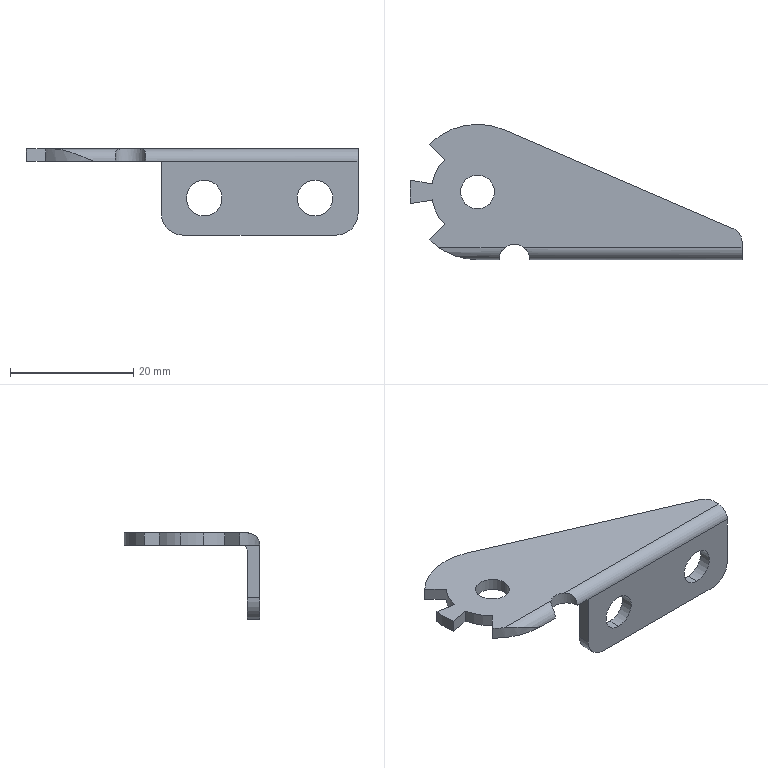Component | SolidWorks | MHPUS204-38-33-A-1_37-1 | 1 solid | 30 faces | box 54 x 22 x 14 mm | volume 2031 mm3 | cylinder 18 | plane 12 | commonest cylinder face diameters 5.8 x4 22 x3 5.5 x2 4 x2 15 x2 7 x2 4.4 x1 5 x1
STEP:
#1=COLOUR_RGB('',0.7922,0.8196,0.9333);
#2=FILL_AREA_STYLE_COLOUR('',#1);
#3=FILL_AREA_STYLE('',(#2));
#4=SURFACE_STYLE_FILL_AREA(#3);
#5=SURFACE_SIDE_STYLE('',(#4));
#6=SURFACE_STYLE_USAGE(.BOTH.,#5);
#7=PRESENTATION_STYLE_ASSIGNMENT((#6));
#8=CARTESIAN_POINT('',(-0.04475,-3.898,3.071));
#9=VERTEX_POINT('',#8);
#10=CARTESIAN_POINT('',(0.1718,-3.898,3.071));
#11=VERTEX_POINT('',#10);
#12=CARTESIAN_POINT('',(0.06352,-3.898,3.071));
#13=DIRECTION('',(0.,0.,1.));
#14=DIRECTION('',(1.,0.,0.));
#15=AXIS2_PLACEMENT_3D('',#12,#13,#14);
#16=CIRCLE('',#15,0.1083);
#17=EDGE_CURVE('',#9,#11,#16,.T.);
#18=ORIENTED_EDGE('',*,*,#17,.F.);
#19=CARTESIAN_POINT('',(-0.04475,-3.898,3.15));
#20=VERTEX_POINT('',#19);
#21=CARTESIAN_POINT('',(-0.04475,-3.898,3.15));
#22=DIRECTION('',(0.,0.,1.));
#23=VECTOR('',#22,39.37);
#24=LINE('',#21,#23);
#25=EDGE_CURVE('',#9,#20,#24,.T.);
#26=ORIENTED_EDGE('',*,*,#25,.T.);
#27=CARTESIAN_POINT('',(0.1718,-3.898,3.15));
#28=VERTEX_POINT('',#27);
#29=CARTESIAN_POINT('',(0.06352,-3.898,3.15));
#30=DIRECTION('',(0.,0.,-1.));
#31=DIRECTION('',(1.,0.,0.));
#32=AXIS2_PLACEMENT_3D('',#29,#30,#31);
#33=CIRCLE('',#32,0.1083);
#34=EDGE_CURVE('',#28,#20,#33,.T.);
#35=ORIENTED_EDGE('',*,*,#34,.F.);
#36=CARTESIAN_POINT('',(0.1718,-3.898,3.15));
#37=DIRECTION('',(0.,0.,1.));
#38=VECTOR('',#37,39.37);
#39=LINE('',#36,#38);
#40=EDGE_CURVE('',#11,#28,#39,.T.);
#41=ORIENTED_EDGE('',*,*,#40,.F.);
#42=EDGE_LOOP('',(#18,#26,#35,#41));
#43=FACE_OUTER_BOUND('',#42,.T.);
#44=CARTESIAN_POINT('',(0.06352,-3.898,3.15));
#45=DIRECTION('',(0.,0.,1.));
#46=DIRECTION('',(1.,0.,0.));
#47=AXIS2_PLACEMENT_3D('',#44,#45,#46);
#48=CYLINDRICAL_SURFACE('',#47,0.1083);
#49=ADVANCED_FACE('',(#43),#48,.F.);
#50=CARTESIAN_POINT('',(0.7722,-4.252,2.72));
#51=VERTEX_POINT('',#50);
#52=CARTESIAN_POINT('',(0.7722,-4.252,2.949));
#53=VERTEX_POINT('',#52);
#54=CARTESIAN_POINT('',(0.7722,-4.252,2.835));
#55=DIRECTION('',(0.,1.,0.));
#56=DIRECTION('',(0.,0.,-1.));
#57=AXIS2_PLACEMENT_3D('',#54,#55,#56);
#58=CIRCLE('',#57,0.1142);
#59=EDGE_CURVE('',#51,#53,#58,.T.);
#60=ORIENTED_EDGE('',*,*,#59,.T.);
#61=CARTESIAN_POINT('',(0.7722,-4.331,2.949));
#62=VERTEX_POINT('',#61);
#63=CARTESIAN_POINT('',(0.7722,-4.331,2.949));
#64=DIRECTION('',(0.,-1.,0.));
#65=VECTOR('',#64,39.37);
#66=LINE('',#63,#65);
#67=EDGE_CURVE('',#53,#62,#66,.T.);
#68=ORIENTED_EDGE('',*,*,#67,.T.);
#69=CARTESIAN_POINT('',(0.7722,-4.331,2.72));
#70=VERTEX_POINT('',#69);
#71=CARTESIAN_POINT('',(0.7722,-4.331,2.835));
#72=DIRECTION('',(0.,1.,0.));
#73=DIRECTION('',(0.,0.,-1.));
#74=AXIS2_PLACEMENT_3D('',#71,#72,#73);
#75=CIRCLE('',#74,0.1142);
#76=EDGE_CURVE('',#70,#62,#75,.T.);
#77=ORIENTED_EDGE('',*,*,#76,.F.);
#78=CARTESIAN_POINT('',(0.7722,-4.331,2.72));
#79=DIRECTION('',(0.,-1.,0.));
#80=VECTOR('',#79,39.37);
#81=LINE('',#78,#80);
#82=EDGE_CURVE('',#51,#70,#81,.T.);
#83=ORIENTED_EDGE('',*,*,#82,.F.);
#84=EDGE_LOOP('',(#60,#68,#77,#83));
#85=FACE_OUTER_BOUND('',#84,.T.);
#86=CARTESIAN_POINT('',(0.7722,-4.331,2.835));
#87=DIRECTION('',(0.,-1.,0.));
#88=DIRECTION('',(0.,0.,-1.));
#89=AXIS2_PLACEMENT_3D('',#86,#87,#88);
#90=CYLINDRICAL_SURFACE('',#89,0.1142);
#91=ADVANCED_FACE('',(#85),#90,.F.);
#92=CARTESIAN_POINT('',(1.481,-4.252,2.72));
#93=VERTEX_POINT('',#92);
#94=CARTESIAN_POINT('',(1.481,-4.252,2.949));
#95=VERTEX_POINT('',#94);
#96=CARTESIAN_POINT('',(1.481,-4.252,2.835));
#97=DIRECTION('',(0.,1.,0.));
#98=DIRECTION('',(0.,0.,-1.));
#99=AXIS2_PLACEMENT_3D('',#96,#97,#98);
#100=CIRCLE('',#99,0.1142);
#101=EDGE_CURVE('',#93,#95,#100,.T.);
#102=ORIENTED_EDGE('',*,*,#101,.T.);
#103=CARTESIAN_POINT('',(1.481,-4.331,2.949));
#104=VERTEX_POINT('',#103);
#105=CARTESIAN_POINT('',(1.481,-4.331,2.949));
#106=DIRECTION('',(0.,-1.,0.));
#107=VECTOR('',#106,39.37);
#108=LINE('',#105,#107);
#109=EDGE_CURVE('',#95,#104,#108,.T.);
#110=ORIENTED_EDGE('',*,*,#109,.T.);
#111=CARTESIAN_POINT('',(1.481,-4.331,2.72));
#112=VERTEX_POINT('',#111);
#113=CARTESIAN_POINT('',(1.481,-4.331,2.835));
#114=DIRECTION('',(0.,1.,0.));
#115=DIRECTION('',(0.,0.,-1.));
#116=AXIS2_PLACEMENT_3D('',#113,#114,#115);
#117=CIRCLE('',#116,0.1142);
#118=EDGE_CURVE('',#112,#104,#117,.T.);
#119=ORIENTED_EDGE('',*,*,#118,.F.);
#120=CARTESIAN_POINT('',(1.481,-4.331,2.72));
#121=DIRECTION('',(0.,-1.,0.));
#122=VECTOR('',#121,39.37);
#123=LINE('',#120,#122);
#124=EDGE_CURVE('',#93,#112,#123,.T.);
#125=ORIENTED_EDGE('',*,*,#124,.F.);
#126=EDGE_LOOP('',(#102,#110,#119,#125));
#127=FACE_OUTER_BOUND('',#126,.T.);
#128=CARTESIAN_POINT('',(1.481,-4.331,2.835));
#129=DIRECTION('',(0.,-1.,0.));
#130=DIRECTION('',(0.,0.,-1.));
#131=AXIS2_PLACEMENT_3D('',#128,#129,#130);
#132=CYLINDRICAL_SURFACE('',#131,0.1142);
#133=ADVANCED_FACE('',(#127),#132,.F.);
#134=ORIENTED_EDGE('',*,*,#34,.T.);
#135=CARTESIAN_POINT('',(0.06352,-3.898,3.15));
#136=DIRECTION('',(0.,0.,-1.));
#137=DIRECTION('',(1.,0.,0.));
#138=AXIS2_PLACEMENT_3D('',#135,#136,#137);
#139=CIRCLE('',#138,0.1083);
#140=EDGE_CURVE('',#20,#28,#139,.T.);
#141=ORIENTED_EDGE('',*,*,#140,.T.);
#142=EDGE_LOOP('',(#134,#141));
#143=FACE_BOUND('',#142,.T.);
#144=CARTESIAN_POINT('',(-0.2427,-4.204,3.15));
#145=VERTEX_POINT('',#144);
#146=CARTESIAN_POINT('',(-0.1855,-4.252,3.15));
#147=VERTEX_POINT('',#146);
#148=CARTESIAN_POINT('',(0.06352,-3.898,3.15));
#149=DIRECTION('',(0.,0.,1.));
#150=DIRECTION('',(1.,0.,0.));
#151=AXIS2_PLACEMENT_3D('',#148,#149,#150);
#152=CIRCLE('',#151,0.4331);
#153=EDGE_CURVE('',#145,#147,#152,.T.);
#154=ORIENTED_EDGE('',*,*,#153,.T.);
#155=CARTESIAN_POINT('',(0.2407,-4.252,3.15));
#156=VERTEX_POINT('',#155);
#157=CARTESIAN_POINT('',(0.06352,-4.252,3.15));
#158=DIRECTION('',(1.,0.,0.));
#159=VECTOR('',#158,39.37);
#160=LINE('',#157,#159);
#161=EDGE_CURVE('',#147,#156,#160,.T.);
#162=ORIENTED_EDGE('',*,*,#161,.T.);
#163=CARTESIAN_POINT('',(0.3588,-4.252,3.15));
#164=VERTEX_POINT('',#163);
#165=CARTESIAN_POINT('',(0.2997,-4.331,3.15));
#166=DIRECTION('',(0.,0.,-1.));
#167=DIRECTION('',(1.,0.,0.));
#168=AXIS2_PLACEMENT_3D('',#165,#166,#167);
#169=CIRCLE('',#168,0.09843);
#170=EDGE_CURVE('',#156,#164,#169,.T.);
#171=ORIENTED_EDGE('',*,*,#170,.T.);
#172=CARTESIAN_POINT('',(1.756,-4.252,3.15));
#173=VERTEX_POINT('',#172);
#174=CARTESIAN_POINT('',(0.06352,-4.252,3.15));
#175=DIRECTION('',(1.,0.,0.));
#176=VECTOR('',#175,39.37);
#177=LINE('',#174,#176);
#178=EDGE_CURVE('',#164,#173,#177,.T.);
#179=ORIENTED_EDGE('',*,*,#178,.T.);
#180=CARTESIAN_POINT('',(1.756,-4.214,3.15));
#181=VERTEX_POINT('',#180);
#182=CARTESIAN_POINT('',(1.756,-4.331,3.15));
#183=DIRECTION('',(0.,-1.,0.));
#184=VECTOR('',#183,39.37);
#185=LINE('',#182,#184);
#186=EDGE_CURVE('',#181,#173,#185,.T.);
#187=ORIENTED_EDGE('',*,*,#186,.F.);
#188=CARTESIAN_POINT('',(1.704,-4.135,3.15));
#189=VERTEX_POINT('',#188);
#190=CARTESIAN_POINT('',(1.67,-4.214,3.15));
#191=DIRECTION('',(0.,0.,1.));
#192=DIRECTION('',(1.,0.,0.));
#193=AXIS2_PLACEMENT_3D('',#190,#191,#192);
#194=CIRCLE('',#193,0.08661);
#195=EDGE_CURVE('',#181,#189,#194,.T.);
#196=ORIENTED_EDGE('',*,*,#195,.T.);
#197=CARTESIAN_POINT('',(0.2353,-3.5,3.15));
#198=VERTEX_POINT('',#197);
#199=CARTESIAN_POINT('',(1.704,-4.135,3.15));
#200=DIRECTION('',(-0.9179,0.3967,0.));
#201=VECTOR('',#200,39.37);
#202=LINE('',#199,#201);
#203=EDGE_CURVE('',#189,#198,#202,.T.);
#204=ORIENTED_EDGE('',*,*,#203,.T.);
#205=CARTESIAN_POINT('',(-0.2427,-3.591,3.15));
#206=VERTEX_POINT('',#205);
#207=CARTESIAN_POINT('',(0.06352,-3.898,3.15));
#208=DIRECTION('',(0.,0.,1.));
#209=DIRECTION('',(1.,0.,0.));
#210=AXIS2_PLACEMENT_3D('',#207,#208,#209);
#211=CIRCLE('',#210,0.4331);
#212=EDGE_CURVE('',#198,#206,#211,.T.);
#213=ORIENTED_EDGE('',*,*,#212,.T.);
#214=CARTESIAN_POINT('',(-0.1453,-3.689,3.15));
#215=VERTEX_POINT('',#214);
#216=CARTESIAN_POINT('',(-0.2427,-3.591,3.15));
#217=DIRECTION('',(0.7071,-0.7071,0.));
#218=VECTOR('',#217,39.37);
#219=LINE('',#216,#218);
#220=EDGE_CURVE('',#206,#215,#219,.T.);
#221=ORIENTED_EDGE('',*,*,#220,.T.);
#222=CARTESIAN_POINT('',(-0.2273,-3.846,3.15));
#223=VERTEX_POINT('',#222);
#224=CARTESIAN_POINT('',(0.06352,-3.898,3.15));
#225=DIRECTION('',(0.,0.,1.));
#226=DIRECTION('',(1.,0.,0.));
#227=AXIS2_PLACEMENT_3D('',#224,#225,#226);
#228=CIRCLE('',#227,0.2953);
#229=EDGE_CURVE('',#215,#223,#228,.T.);
#230=ORIENTED_EDGE('',*,*,#229,.T.);
#231=CARTESIAN_POINT('',(-0.363,-3.822,3.15));
#232=VERTEX_POINT('',#231);
#233=CARTESIAN_POINT('',(-0.2273,-3.846,3.15));
#234=DIRECTION('',(-0.9848,0.1736,0.));
#235=VECTOR('',#234,39.37);
#236=LINE('',#233,#235);
#237=EDGE_CURVE('',#223,#232,#236,.T.);
#238=ORIENTED_EDGE('',*,*,#237,.T.);
#239=CARTESIAN_POINT('',(-0.363,-3.973,3.15));
#240=VERTEX_POINT('',#239);
#241=CARTESIAN_POINT('',(0.06352,-3.898,3.15));
#242=DIRECTION('',(0.,0.,1.));
#243=DIRECTION('',(1.,0.,0.));
#244=AXIS2_PLACEMENT_3D('',#241,#242,#243);
#245=CIRCLE('',#244,0.4331);
#246=EDGE_CURVE('',#232,#240,#245,.T.);
#247=ORIENTED_EDGE('',*,*,#246,.T.);
#248=CARTESIAN_POINT('',(-0.2273,-3.949,3.15));
#249=VERTEX_POINT('',#248);
#250=CARTESIAN_POINT('',(-0.363,-3.973,3.15));
#251=DIRECTION('',(0.9848,0.1736,0.));
#252=VECTOR('',#251,39.37);
#253=LINE('',#250,#252);
#254=EDGE_CURVE('',#240,#249,#253,.T.);
#255=ORIENTED_EDGE('',*,*,#254,.T.);
#256=CARTESIAN_POINT('',(-0.1453,-4.106,3.15));
#257=VERTEX_POINT('',#256);
#258=CARTESIAN_POINT('',(0.06352,-3.898,3.15));
#259=DIRECTION('',(0.,0.,1.));
#260=DIRECTION('',(1.,0.,0.));
#261=AXIS2_PLACEMENT_3D('',#258,#259,#260);
#262=CIRCLE('',#261,0.2953);
#263=EDGE_CURVE('',#249,#257,#262,.T.);
#264=ORIENTED_EDGE('',*,*,#263,.T.);
#265=CARTESIAN_POINT('',(-0.1453,-4.106,3.15));
#266=DIRECTION('',(-0.7071,-0.7071,0.));
#267=VECTOR('',#266,39.37);
#268=LINE('',#265,#267);
#269=EDGE_CURVE('',#257,#145,#268,.T.);
#270=ORIENTED_EDGE('',*,*,#269,.T.);
#271=EDGE_LOOP('',(#154,#162,#171,#179,#187,#196,#204,#213,#221,#230,#238,#247,#255,#264,#270));
#272=FACE_OUTER_BOUND('',#271,.T.);
#273=CARTESIAN_POINT('',(0.06352,-4.331,3.15));
#274=DIRECTION('',(0.,0.,1.));
#275=DIRECTION('',(1.,0.,0.));
#276=AXIS2_PLACEMENT_3D('',#273,#274,#275);
#277=PLANE('',#276);
#278=ADVANCED_FACE('',(#143,#272),#277,.T.);
#279=ORIENTED_EDGE('',*,*,#25,.F.);
#280=CARTESIAN_POINT('',(0.06352,-3.898,3.071));
#281=DIRECTION('',(0.,0.,1.));
#282=DIRECTION('',(1.,0.,0.));
#283=AXIS2_PLACEMENT_3D('',#280,#281,#282);
#284=CIRCLE('',#283,0.1083);
#285=EDGE_CURVE('',#11,#9,#284,.T.);
#286=ORIENTED_EDGE('',*,*,#285,.F.);
#287=ORIENTED_EDGE('',*,*,#40,.T.);
#288=ORIENTED_EDGE('',*,*,#140,.F.);
#289=EDGE_LOOP('',(#279,#286,#287,#288));
#290=FACE_OUTER_BOUND('',#289,.T.);
#291=CARTESIAN_POINT('',(0.06352,-3.898,3.15));
#292=DIRECTION('',(0.,0.,1.));
#293=DIRECTION('',(1.,0.,0.));
#294=AXIS2_PLACEMENT_3D('',#291,#292,#293);
#295=CYLINDRICAL_SURFACE('',#294,0.1083);
#296=ADVANCED_FACE('',(#290),#295,.F.);
#297=CARTESIAN_POINT('',(0.06352,-4.331,3.071));
#298=VERTEX_POINT('',#297);
#299=CARTESIAN_POINT('',(-0.1855,-4.252,3.15));
#300=CARTESIAN_POINT('',(-0.1663,-4.265,3.15));
#301=CARTESIAN_POINT('',(-0.1465,-4.277,3.146));
#302=CARTESIAN_POINT('',(-0.1158,-4.292,3.139));
#303=CARTESIAN_POINT('',(-0.1054,-4.297,3.136));
#304=CARTESIAN_POINT('',(-0.08469,-4.305,3.13));
#305=CARTESIAN_POINT('',(-0.0743,-4.308,3.126));
#306=CARTESIAN_POINT('',(-0.04301,-4.318,3.115));
#307=CARTESIAN_POINT('',(-0.02197,-4.323,3.107));
#308=CARTESIAN_POINT('',(0.01002,-4.328,3.094));
#309=CARTESIAN_POINT('',(0.02072,-4.329,3.089));
#310=CARTESIAN_POINT('',(0.0421,-4.33,3.08));
#311=CARTESIAN_POINT('',(0.05286,-4.331,3.075));
#312=CARTESIAN_POINT('',(0.06352,-4.331,3.071));
#313=B_SPLINE_CURVE_WITH_KNOTS('',3,(#299,#300,#301,#302,#303,#304,#305,#306,#307,#308,#309,#310,#311,#312),.UNSPECIFIED.,.F.,.F.,(4,2,2,2,2,2,4),(0.,0.001765,0.002648,0.003531,0.005296,0.006179,0.007061),.UNSPECIFIED.);
#314=EDGE_CURVE('',#147,#298,#313,.T.);
#315=ORIENTED_EDGE('',*,*,#314,.T.);
#316=CARTESIAN_POINT('',(0.2013,-4.331,3.071));
#317=VERTEX_POINT('',#316);
#318=CARTESIAN_POINT('',(1.756,-4.331,3.071));
#319=DIRECTION('',(1.,0.,0.));
#320=VECTOR('',#319,39.37);
#321=LINE('',#318,#320);
#322=EDGE_CURVE('',#298,#317,#321,.T.);
#323=ORIENTED_EDGE('',*,*,#322,.T.);
#324=CARTESIAN_POINT('',(0.2013,-4.331,3.071));
#325=CARTESIAN_POINT('',(0.2013,-4.331,3.077));
#326=CARTESIAN_POINT('',(0.2013,-4.33,3.082));
#327=CARTESIAN_POINT('',(0.2013,-4.328,3.093));
#328=CARTESIAN_POINT('',(0.2014,-4.326,3.099));
#329=CARTESIAN_POINT('',(0.2017,-4.321,3.109));
#330=CARTESIAN_POINT('',(0.202,-4.318,3.114));
#331=CARTESIAN_POINT('',(0.2031,-4.311,3.123));
#332=CARTESIAN_POINT('',(0.204,-4.308,3.127));
#333=CARTESIAN_POINT('',(0.2063,-4.299,3.134));
#334=CARTESIAN_POINT('',(0.208,-4.295,3.137));
#335=CARTESIAN_POINT('',(0.2121,-4.286,3.142));
#336=CARTESIAN_POINT('',(0.2146,-4.281,3.144));
#337=CARTESIAN_POINT('',(0.2237,-4.267,3.149));
#338=CARTESIAN_POINT('',(0.2316,-4.259,3.15));
#339=CARTESIAN_POINT('',(0.2407,-4.252,3.15));
#340=B_SPLINE_CURVE_WITH_KNOTS('',3,(#324,#325,#326,#327,#328,#329,#330,#331,#332,#333,#334,#335,#336,#337,#338,#339),.UNSPECIFIED.,.F.,.F.,(4,2,2,2,2,2,2,4),(0.,0.0004284,0.0008569,0.001285,0.001714,0.002142,0.002571,0.003428),.UNSPECIFIED.);
#341=EDGE_CURVE('',#317,#156,#340,.T.);
#342=ORIENTED_EDGE('',*,*,#341,.T.);
#343=ORIENTED_EDGE('',*,*,#161,.F.);
#344=EDGE_LOOP('',(#315,#323,#342,#343));
#345=FACE_OUTER_BOUND('',#344,.T.);
#346=CARTESIAN_POINT('',(1.756,-4.252,3.071));
#347=DIRECTION('',(1.,0.,0.));
#348=DIRECTION('',(0.,0.,-1.));
#349=AXIS2_PLACEMENT_3D('',#346,#347,#348);
#350=CYLINDRICAL_SURFACE('',#349,0.07874);
#351=ADVANCED_FACE('',(#345),#350,.T.);
#352=ORIENTED_EDGE('',*,*,#153,.F.);
#353=CARTESIAN_POINT('',(-0.2427,-4.204,3.071));
#354=VERTEX_POINT('',#353);
#355=CARTESIAN_POINT('',(-0.2427,-4.204,3.15));
#356=DIRECTION('',(0.,0.,-1.));
#357=VECTOR('',#356,39.37);
#358=LINE('',#355,#357);
#359=EDGE_CURVE('',#145,#354,#358,.T.);
#360=ORIENTED_EDGE('',*,*,#359,.T.);
#361=CARTESIAN_POINT('',(0.06352,-3.898,3.071));
#362=DIRECTION('',(0.,0.,1.));
#363=DIRECTION('',(1.,0.,0.));
#364=AXIS2_PLACEMENT_3D('',#361,#362,#363);
#365=CIRCLE('',#364,0.4331);
#366=EDGE_CURVE('',#354,#298,#365,.T.);
#367=ORIENTED_EDGE('',*,*,#366,.T.);
#368=ORIENTED_EDGE('',*,*,#314,.F.);
#369=EDGE_LOOP('',(#352,#360,#367,#368));
#370=FACE_OUTER_BOUND('',#369,.T.);
#371=CARTESIAN_POINT('',(0.06352,-3.898,3.15));
#372=DIRECTION('',(0.,0.,1.));
#373=DIRECTION('',(1.,0.,0.));
#374=AXIS2_PLACEMENT_3D('',#371,#372,#373);
#375=CYLINDRICAL_SURFACE('',#374,0.4331);
#376=ADVANCED_FACE('',(#370),#375,.T.);
#377=ORIENTED_EDGE('',*,*,#269,.F.);
#378=CARTESIAN_POINT('',(-0.1453,-4.106,3.071));
#379=VERTEX_POINT('',#378);
#380=CARTESIAN_POINT('',(-0.1453,-4.106,3.15));
#381=DIRECTION('',(0.,0.,-1.));
#382=VECTOR('',#381,39.37);
#383=LINE('',#380,#382);
#384=EDGE_CURVE('',#257,#379,#383,.T.);
#385=ORIENTED_EDGE('',*,*,#384,.T.);
#386=CARTESIAN_POINT('',(-0.1453,-4.106,3.071));
#387=DIRECTION('',(-0.7071,-0.7071,0.));
#388=VECTOR('',#387,39.37);
#389=LINE('',#386,#388);
#390=EDGE_CURVE('',#379,#354,#389,.T.);
#391=ORIENTED_EDGE('',*,*,#390,.T.);
#392=ORIENTED_EDGE('',*,*,#359,.F.);
#393=EDGE_LOOP('',(#377,#385,#391,#392));
#394=FACE_OUTER_BOUND('',#393,.T.);
#395=CARTESIAN_POINT('',(-0.1453,-4.106,3.15));
#396=DIRECTION('',(-0.7071,0.7071,0.));
#397=DIRECTION('',(-0.7071,-0.7071,0.));
#398=AXIS2_PLACEMENT_3D('',#395,#396,#397);
#399=PLANE('',#398);
#400=ADVANCED_FACE('',(#394),#399,.T.);
#401=ORIENTED_EDGE('',*,*,#263,.F.);
#402=CARTESIAN_POINT('',(-0.2273,-3.949,3.071));
#403=VERTEX_POINT('',#402);
#404=CARTESIAN_POINT('',(-0.2273,-3.949,3.15));
#405=DIRECTION('',(0.,0.,-1.));
#406=VECTOR('',#405,39.37);
#407=LINE('',#404,#406);
#408=EDGE_CURVE('',#249,#403,#407,.T.);
#409=ORIENTED_EDGE('',*,*,#408,.T.);
#410=CARTESIAN_POINT('',(0.06352,-3.898,3.071));
#411=DIRECTION('',(0.,0.,1.));
#412=DIRECTION('',(1.,0.,0.));
#413=AXIS2_PLACEMENT_3D('',#410,#411,#412);
#414=CIRCLE('',#413,0.2953);
#415=EDGE_CURVE('',#403,#379,#414,.T.);
#416=ORIENTED_EDGE('',*,*,#415,.T.);
#417=ORIENTED_EDGE('',*,*,#384,.F.);
#418=EDGE_LOOP('',(#401,#409,#416,#417));
#419=FACE_OUTER_BOUND('',#418,.T.);
#420=CARTESIAN_POINT('',(0.06352,-3.898,3.15));
#421=DIRECTION('',(0.,0.,1.));
#422=DIRECTION('',(1.,0.,0.));
#423=AXIS2_PLACEMENT_3D('',#420,#421,#422);
#424=CYLINDRICAL_SURFACE('',#423,0.2953);
#425=ADVANCED_FACE('',(#419),#424,.T.);
#426=ORIENTED_EDGE('',*,*,#254,.F.);
#427=CARTESIAN_POINT('',(-0.363,-3.973,3.071));
#428=VERTEX_POINT('',#427);
#429=CARTESIAN_POINT('',(-0.363,-3.973,3.15));
#430=DIRECTION('',(0.,0.,-1.));
#431=VECTOR('',#430,39.37);
#432=LINE('',#429,#431);
#433=EDGE_CURVE('',#240,#428,#432,.T.);
#434=ORIENTED_EDGE('',*,*,#433,.T.);
#435=CARTESIAN_POINT('',(-0.363,-3.973,3.071));
#436=DIRECTION('',(0.9848,0.1736,0.));
#437=VECTOR('',#436,39.37);
#438=LINE('',#435,#437);
#439=EDGE_CURVE('',#428,#403,#438,.T.);
#440=ORIENTED_EDGE('',*,*,#439,.T.);
#441=ORIENTED_EDGE('',*,*,#408,.F.);
#442=EDGE_LOOP('',(#426,#434,#440,#441));
#443=FACE_OUTER_BOUND('',#442,.T.);
#444=CARTESIAN_POINT('',(-0.363,-3.973,3.15));
#445=DIRECTION('',(0.1736,-0.9848,0.));
#446=DIRECTION('',(0.9848,0.1736,0.));
#447=AXIS2_PLACEMENT_3D('',#444,#445,#446);
#448=PLANE('',#447);
#449=ADVANCED_FACE('',(#443),#448,.T.);
#450=ORIENTED_EDGE('',*,*,#246,.F.);
#451=CARTESIAN_POINT('',(-0.363,-3.822,3.071));
#452=VERTEX_POINT('',#451);
#453=CARTESIAN_POINT('',(-0.363,-3.822,3.15));
#454=DIRECTION('',(0.,0.,-1.));
#455=VECTOR('',#454,39.37);
#456=LINE('',#453,#455);
#457=EDGE_CURVE('',#232,#452,#456,.T.);
#458=ORIENTED_EDGE('',*,*,#457,.T.);
#459=CARTESIAN_POINT('',(0.06352,-3.898,3.071));
#460=DIRECTION('',(0.,0.,1.));
#461=DIRECTION('',(1.,0.,0.));
#462=AXIS2_PLACEMENT_3D('',#459,#460,#461);
#463=CIRCLE('',#462,0.4331);
#464=EDGE_CURVE('',#452,#428,#463,.T.);
#465=ORIENTED_EDGE('',*,*,#464,.T.);
#466=ORIENTED_EDGE('',*,*,#433,.F.);
#467=EDGE_LOOP('',(#450,#458,#465,#466));
#468=FACE_OUTER_BOUND('',#467,.T.);
#469=CARTESIAN_POINT('',(0.06352,-3.898,3.15));
#470=DIRECTION('',(0.,0.,1.));
#471=DIRECTION('',(1.,0.,0.));
#472=AXIS2_PLACEMENT_3D('',#469,#470,#471);
#473=CYLINDRICAL_SURFACE('',#472,0.4331);
#474=ADVANCED_FACE('',(#468),#473,.T.);
#475=ORIENTED_EDGE('',*,*,#237,.F.);
#476=CARTESIAN_POINT('',(-0.2273,-3.846,3.071));
#477=VERTEX_POINT('',#476);
#478=CARTESIAN_POINT('',(-0.2273,-3.846,3.15));
#479=DIRECTION('',(0.,0.,-1.));
#480=VECTOR('',#479,39.37);
#481=LINE('',#478,#480);
#482=EDGE_CURVE('',#223,#477,#481,.T.);
#483=ORIENTED_EDGE('',*,*,#482,.T.);
#484=CARTESIAN_POINT('',(-0.2273,-3.846,3.071));
#485=DIRECTION('',(-0.9848,0.1736,0.));
#486=VECTOR('',#485,39.37);
#487=LINE('',#484,#486);
#488=EDGE_CURVE('',#477,#452,#487,.T.);
#489=ORIENTED_EDGE('',*,*,#488,.T.);
#490=ORIENTED_EDGE('',*,*,#457,.F.);
#491=EDGE_LOOP('',(#475,#483,#489,#490));
#492=FACE_OUTER_BOUND('',#491,.T.);
#493=CARTESIAN_POINT('',(-0.2273,-3.846,3.15));
#494=DIRECTION('',(0.1736,0.9848,0.));
#495=DIRECTION('',(-0.9848,0.1736,0.));
#496=AXIS2_PLACEMENT_3D('',#493,#494,#495);
#497=PLANE('',#496);
#498=ADVANCED_FACE('',(#492),#497,.T.);
#499=ORIENTED_EDGE('',*,*,#229,.F.);
#500=CARTESIAN_POINT('',(-0.1453,-3.689,3.071));
#501=VERTEX_POINT('',#500);
#502=CARTESIAN_POINT('',(-0.1453,-3.689,3.15));
#503=DIRECTION('',(0.,0.,-1.));
#504=VECTOR('',#503,39.37);
#505=LINE('',#502,#504);
#506=EDGE_CURVE('',#215,#501,#505,.T.);
#507=ORIENTED_EDGE('',*,*,#506,.T.);
#508=CARTESIAN_POINT('',(0.06352,-3.898,3.071));
#509=DIRECTION('',(0.,0.,1.));
#510=DIRECTION('',(1.,0.,0.));
#511=AXIS2_PLACEMENT_3D('',#508,#509,#510);
#512=CIRCLE('',#511,0.2953);
#513=EDGE_CURVE('',#501,#477,#512,.T.);
#514=ORIENTED_EDGE('',*,*,#513,.T.);
#515=ORIENTED_EDGE('',*,*,#482,.F.);
#516=EDGE_LOOP('',(#499,#507,#514,#515));
#517=FACE_OUTER_BOUND('',#516,.T.);
#518=CARTESIAN_POINT('',(0.06352,-3.898,3.15));
#519=DIRECTION('',(0.,0.,1.));
#520=DIRECTION('',(1.,0.,0.));
#521=AXIS2_PLACEMENT_3D('',#518,#519,#520);
#522=CYLINDRICAL_SURFACE('',#521,0.2953);
#523=ADVANCED_FACE('',(#517),#522,.T.);
#524=ORIENTED_EDGE('',*,*,#220,.F.);
#525=CARTESIAN_POINT('',(-0.2427,-3.591,3.071));
#526=VERTEX_POINT('',#525);
#527=CARTESIAN_POINT('',(-0.2427,-3.591,3.15));
#528=DIRECTION('',(0.,0.,-1.));
#529=VECTOR('',#528,39.37);
#530=LINE('',#527,#529);
#531=EDGE_CURVE('',#206,#526,#530,.T.);
#532=ORIENTED_EDGE('',*,*,#531,.T.);
#533=CARTESIAN_POINT('',(-0.2427,-3.591,3.071));
#534=DIRECTION('',(0.7071,-0.7071,0.));
#535=VECTOR('',#534,39.37);
#536=LINE('',#533,#535);
#537=EDGE_CURVE('',#526,#501,#536,.T.);
#538=ORIENTED_EDGE('',*,*,#537,.T.);
#539=ORIENTED_EDGE('',*,*,#506,.F.);
#540=EDGE_LOOP('',(#524,#532,#538,#539));
#541=FACE_OUTER_BOUND('',#540,.T.);
#542=CARTESIAN_POINT('',(-0.2427,-3.591,3.15));
#543=DIRECTION('',(-0.7071,-0.7071,0.));
#544=DIRECTION('',(0.7071,-0.7071,0.));
#545=AXIS2_PLACEMENT_3D('',#542,#543,#544);
#546=PLANE('',#545);
#547=ADVANCED_FACE('',(#541),#546,.T.);
#548=ORIENTED_EDGE('',*,*,#212,.F.);
#549=CARTESIAN_POINT('',(0.2353,-3.5,3.071));
#550=VERTEX_POINT('',#549);
#551=CARTESIAN_POINT('',(0.2353,-3.5,3.15));
#552=DIRECTION('',(0.,0.,-1.));
#553=VECTOR('',#552,39.37);
#554=LINE('',#551,#553);
#555=EDGE_CURVE('',#198,#550,#554,.T.);
#556=ORIENTED_EDGE('',*,*,#555,.T.);
#557=CARTESIAN_POINT('',(0.06352,-3.898,3.071));
#558=DIRECTION('',(0.,0.,1.));
#559=DIRECTION('',(1.,0.,0.));
#560=AXIS2_PLACEMENT_3D('',#557,#558,#559);
#561=CIRCLE('',#560,0.4331);
#562=EDGE_CURVE('',#550,#526,#561,.T.);
#563=ORIENTED_EDGE('',*,*,#562,.T.);
#564=ORIENTED_EDGE('',*,*,#531,.F.);
#565=EDGE_LOOP('',(#548,#556,#563,#564));
#566=FACE_OUTER_BOUND('',#565,.T.);
#567=CARTESIAN_POINT('',(0.06352,-3.898,3.15));
#568=DIRECTION('',(0.,0.,1.));
#569=DIRECTION('',(1.,0.,0.));
#570=AXIS2_PLACEMENT_3D('',#567,#568,#569);
#571=CYLINDRICAL_SURFACE('',#570,0.4331);
#572=ADVANCED_FACE('',(#566),#571,.T.);
#573=ORIENTED_EDGE('',*,*,#203,.F.);
#574=CARTESIAN_POINT('',(1.704,-4.135,3.071));
#575=VERTEX_POINT('',#574);
#576=CARTESIAN_POINT('',(1.704,-4.135,3.15));
#577=DIRECTION('',(0.,0.,-1.));
#578=VECTOR('',#577,39.37);
#579=LINE('',#576,#578);
#580=EDGE_CURVE('',#189,#575,#579,.T.);
#581=ORIENTED_EDGE('',*,*,#580,.T.);
#582=CARTESIAN_POINT('',(1.704,-4.135,3.071));
#583=DIRECTION('',(-0.9179,0.3967,0.));
#584=VECTOR('',#583,39.37);
#585=LINE('',#582,#584);
#586=EDGE_CURVE('',#575,#550,#585,.T.);
#587=ORIENTED_EDGE('',*,*,#586,.T.);
#588=ORIENTED_EDGE('',*,*,#555,.F.);
#589=EDGE_LOOP('',(#573,#581,#587,#588));
#590=FACE_OUTER_BOUND('',#589,.T.);
#591=CARTESIAN_POINT('',(1.704,-4.135,3.15));
#592=DIRECTION('',(0.3967,0.9179,0.));
#593=DIRECTION('',(-0.9179,0.3967,0.));
#594=AXIS2_PLACEMENT_3D('',#591,#592,#593);
#595=PLANE('',#594);
#596=ADVANCED_FACE('',(#590),#595,.T.);
#597=ORIENTED_EDGE('',*,*,#195,.F.);
#598=CARTESIAN_POINT('',(1.756,-4.214,3.071));
#599=VERTEX_POINT('',#598);
#600=CARTESIAN_POINT('',(1.756,-4.214,3.15));
#601=DIRECTION('',(0.,0.,-1.));
#602=VECTOR('',#601,39.37);
#603=LINE('',#600,#602);
#604=EDGE_CURVE('',#181,#599,#603,.T.);
#605=ORIENTED_EDGE('',*,*,#604,.T.);
#606=CARTESIAN_POINT('',(1.756,-4.213,3.071));
#607=VERTEX_POINT('',#606);
#608=CARTESIAN_POINT('',(1.756,-4.214,3.071));
#609=CARTESIAN_POINT('',(1.756,-4.214,3.071));
#610=CARTESIAN_POINT('',(1.756,-4.213,3.071));
#611=CARTESIAN_POINT('',(1.756,-4.213,3.071));
#612=B_SPLINE_CURVE_WITH_KNOTS('',3,(#608,#609,#610,#611),.UNSPECIFIED.,.F.,.F.,(4,4),(0.,0.0000459),.UNSPECIFIED.);
#613=EDGE_CURVE('',#599,#607,#612,.T.);
#614=ORIENTED_EDGE('',*,*,#613,.T.);
#615=CARTESIAN_POINT('',(1.67,-4.214,3.071));
#616=DIRECTION('',(0.,0.,1.));
#617=DIRECTION('',(1.,0.,0.));
#618=AXIS2_PLACEMENT_3D('',#615,#616,#617);
#619=CIRCLE('',#618,0.08661);
#620=EDGE_CURVE('',#607,#575,#619,.T.);
#621=ORIENTED_EDGE('',*,*,#620,.T.);
#622=ORIENTED_EDGE('',*,*,#580,.F.);
#623=EDGE_LOOP('',(#597,#605,#614,#621,#622));
#624=FACE_OUTER_BOUND('',#623,.T.);
#625=CARTESIAN_POINT('',(1.67,-4.214,3.15));
#626=DIRECTION('',(0.,0.,1.));
#627=DIRECTION('',(1.,0.,0.));
#628=AXIS2_PLACEMENT_3D('',#625,#626,#627);
#629=CYLINDRICAL_SURFACE('',#628,0.08661);
#630=ADVANCED_FACE('',(#624),#629,.T.);
#631=CARTESIAN_POINT('',(1.756,-4.331,3.071));
#632=VERTEX_POINT('',#631);
#633=CARTESIAN_POINT('',(1.756,-4.252,3.071));
#634=DIRECTION('',(-1.,0.,0.));
#635=DIRECTION('',(0.,0.,-1.));
#636=AXIS2_PLACEMENT_3D('',#633,#634,#635);
#637=CIRCLE('',#636,0.07874);
#638=EDGE_CURVE('',#632,#173,#637,.T.);
#639=ORIENTED_EDGE('',*,*,#638,.T.);
#640=ORIENTED_EDGE('',*,*,#178,.F.);
#641=CARTESIAN_POINT('',(0.3982,-4.331,3.071));
#642=VERTEX_POINT('',#641);
#643=CARTESIAN_POINT('',(0.3588,-4.252,3.15));
#644=CARTESIAN_POINT('',(0.3633,-4.255,3.15));
#645=CARTESIAN_POINT('',(0.3675,-4.259,3.149));
#646=CARTESIAN_POINT('',(0.3752,-4.267,3.148));
#647=CARTESIAN_POINT('',(0.3787,-4.272,3.147));
#648=CARTESIAN_POINT('',(0.3847,-4.281,3.144));
#649=CARTESIAN_POINT('',(0.3873,-4.285,3.142));
#650=CARTESIAN_POINT('',(0.3915,-4.295,3.137));
#651=CARTESIAN_POINT('',(0.3931,-4.299,3.134));
#652=CARTESIAN_POINT('',(0.3955,-4.307,3.127));
#653=CARTESIAN_POINT('',(0.3963,-4.311,3.123));
#654=CARTESIAN_POINT('',(0.3974,-4.318,3.114));
#655=CARTESIAN_POINT('',(0.3977,-4.321,3.109));
#656=CARTESIAN_POINT('',(0.3981,-4.326,3.099));
#657=CARTESIAN_POINT('',(0.3981,-4.328,3.093));
#658=CARTESIAN_POINT('',(0.3982,-4.33,3.082));
#659=CARTESIAN_POINT('',(0.3982,-4.331,3.077));
#660=CARTESIAN_POINT('',(0.3982,-4.331,3.071));
#661=B_SPLINE_CURVE_WITH_KNOTS('',3,(#643,#644,#645,#646,#647,#648,#649,#650,#651,#652,#653,#654,#655,#656,#657,#658,#659,#660),.UNSPECIFIED.,.F.,.F.,(4,2,2,2,2,2,2,2,4),(0.,0.0004287,0.0008574,0.001286,0.001715,0.002144,0.002572,0.003001,0.00343),.UNSPECIFIED.);
#662=EDGE_CURVE('',#164,#642,#661,.T.);
#663=ORIENTED_EDGE('',*,*,#662,.T.);
#664=CARTESIAN_POINT('',(0.4966,-4.331,3.071));
#665=VERTEX_POINT('',#664);
#666=CARTESIAN_POINT('',(1.756,-4.331,3.071));
#667=DIRECTION('',(1.,0.,0.));
#668=VECTOR('',#667,39.37);
#669=LINE('',#666,#668);
#670=EDGE_CURVE('',#642,#665,#669,.T.);
#671=ORIENTED_EDGE('',*,*,#670,.T.);
#672=CARTESIAN_POINT('',(1.756,-4.331,3.071));
#673=DIRECTION('',(1.,0.,0.));
#674=VECTOR('',#673,39.37);
#675=LINE('',#672,#674);
#676=EDGE_CURVE('',#665,#632,#675,.T.);
#677=ORIENTED_EDGE('',*,*,#676,.T.);
#678=EDGE_LOOP('',(#639,#640,#663,#671,#677));
#679=FACE_OUTER_BOUND('',#678,.T.);
#680=CARTESIAN_POINT('',(1.756,-4.252,3.071));
#681=DIRECTION('',(1.,0.,0.));
#682=DIRECTION('',(0.,0.,-1.));
#683=AXIS2_PLACEMENT_3D('',#680,#681,#682);
#684=CYLINDRICAL_SURFACE('',#683,0.07874);
#685=ADVANCED_FACE('',(#679),#684,.T.);
#686=ORIENTED_EDGE('',*,*,#170,.F.);
#687=ORIENTED_EDGE('',*,*,#341,.F.);
#688=CARTESIAN_POINT('',(0.2997,-4.331,3.071));
#689=DIRECTION('',(0.,0.,1.));
#690=DIRECTION('',(1.,0.,0.));
#691=AXIS2_PLACEMENT_3D('',#688,#689,#690);
#692=CIRCLE('',#691,0.09843);
#693=EDGE_CURVE('',#642,#317,#692,.T.);
#694=ORIENTED_EDGE('',*,*,#693,.F.);
#695=ORIENTED_EDGE('',*,*,#662,.F.);
#696=EDGE_LOOP('',(#686,#687,#694,#695));
#697=FACE_OUTER_BOUND('',#696,.T.);
#698=CARTESIAN_POINT('',(0.2997,-4.331,3.15));
#699=DIRECTION('',(0.,0.,1.));
#700=DIRECTION('',(1.,0.,0.));
#701=AXIS2_PLACEMENT_3D('',#698,#699,#700);
#702=CYLINDRICAL_SURFACE('',#701,0.09843);
#703=ADVANCED_FACE('',(#697),#702,.F.);
#704=ORIENTED_EDGE('',*,*,#285,.T.);
#705=ORIENTED_EDGE('',*,*,#17,.T.);
#706=EDGE_LOOP('',(#704,#705));
#707=FACE_BOUND('',#706,.T.);
#708=ORIENTED_EDGE('',*,*,#322,.F.);
#709=ORIENTED_EDGE('',*,*,#366,.F.);
#710=ORIENTED_EDGE('',*,*,#390,.F.);
#711=ORIENTED_EDGE('',*,*,#415,.F.);
#712=ORIENTED_EDGE('',*,*,#439,.F.);
#713=ORIENTED_EDGE('',*,*,#464,.F.);
#714=ORIENTED_EDGE('',*,*,#488,.F.);
#715=ORIENTED_EDGE('',*,*,#513,.F.);
#716=ORIENTED_EDGE('',*,*,#537,.F.);
#717=ORIENTED_EDGE('',*,*,#562,.F.);
#718=ORIENTED_EDGE('',*,*,#586,.F.);
#719=ORIENTED_EDGE('',*,*,#620,.F.);
#720=CARTESIAN_POINT('',(0.4966,-4.213,3.071));
#721=VERTEX_POINT('',#720);
#722=CARTESIAN_POINT('',(1.756,-4.213,3.071));
#723=DIRECTION('',(1.,0.,0.));
#724=VECTOR('',#723,39.37);
#725=LINE('',#722,#724);
#726=EDGE_CURVE('',#721,#607,#725,.T.);
#727=ORIENTED_EDGE('',*,*,#726,.F.);
#728=CARTESIAN_POINT('',(0.4966,-3.465,3.071));
#729=DIRECTION('',(0.,1.,0.));
#730=VECTOR('',#729,39.37);
#731=LINE('',#728,#730);
#732=EDGE_CURVE('',#665,#721,#731,.T.);
#733=ORIENTED_EDGE('',*,*,#732,.F.);
#734=ORIENTED_EDGE('',*,*,#670,.F.);
#735=ORIENTED_EDGE('',*,*,#693,.T.);
#736=EDGE_LOOP('',(#708,#709,#710,#711,#712,#713,#714,#715,#716,#717,#718,#719,#727,#733,#734,#735));
#737=FACE_OUTER_BOUND('',#736,.T.);
#738=CARTESIAN_POINT('',(1.756,-3.465,3.071));
#739=DIRECTION('',(0.,0.,1.));
#740=DIRECTION('',(1.,0.,0.));
#741=AXIS2_PLACEMENT_3D('',#738,#739,#740);
#742=PLANE('',#741);
#743=ADVANCED_FACE('',(#707,#737),#742,.F.);
#744=ORIENTED_EDGE('',*,*,#638,.F.);
#745=CARTESIAN_POINT('',(1.756,-4.331,2.736));
#746=VERTEX_POINT('',#745);
#747=CARTESIAN_POINT('',(1.756,-4.331,3.15));
#748=DIRECTION('',(0.,0.,-1.));
#749=VECTOR('',#748,39.37);
#750=LINE('',#747,#749);
#751=EDGE_CURVE('',#632,#746,#750,.T.);
#752=ORIENTED_EDGE('',*,*,#751,.T.);
#753=CARTESIAN_POINT('',(1.756,-4.252,2.736));
#754=VERTEX_POINT('',#753);
#755=CARTESIAN_POINT('',(1.756,-4.331,2.736));
#756=DIRECTION('',(0.,1.,0.));
#757=VECTOR('',#756,39.37);
#758=LINE('',#755,#757);
#759=EDGE_CURVE('',#746,#754,#758,.T.);
#760=ORIENTED_EDGE('',*,*,#759,.T.);
#761=CARTESIAN_POINT('',(1.756,-4.252,3.031));
#762=VERTEX_POINT('',#761);
#763=CARTESIAN_POINT('',(1.756,-4.252,3.15));
#764=DIRECTION('',(0.,0.,1.));
#765=VECTOR('',#764,39.37);
#766=LINE('',#763,#765);
#767=EDGE_CURVE('',#754,#762,#766,.T.);
#768=ORIENTED_EDGE('',*,*,#767,.T.);
#769=CARTESIAN_POINT('',(1.756,-4.213,3.031));
#770=DIRECTION('',(-1.,0.,0.));
#771=DIRECTION('',(0.,0.,-1.));
#772=AXIS2_PLACEMENT_3D('',#769,#770,#771);
#773=CIRCLE('',#772,0.03937);
#774=EDGE_CURVE('',#762,#599,#773,.T.);
#775=ORIENTED_EDGE('',*,*,#774,.T.);
#776=ORIENTED_EDGE('',*,*,#604,.F.);
#777=ORIENTED_EDGE('',*,*,#186,.T.);
#778=EDGE_LOOP('',(#744,#752,#760,#768,#775,#776,#777));
#779=FACE_OUTER_BOUND('',#778,.T.);
#780=CARTESIAN_POINT('',(1.756,-4.331,3.15));
#781=DIRECTION('',(1.,0.,0.));
#782=DIRECTION('',(0.,0.,-1.));
#783=AXIS2_PLACEMENT_3D('',#780,#781,#782);
#784=PLANE('',#783);
#785=ADVANCED_FACE('',(#779),#784,.T.);
#786=CARTESIAN_POINT('',(0.4966,-4.331,2.736));
#787=VERTEX_POINT('',#786);
#788=CARTESIAN_POINT('',(0.6344,-4.331,2.598));
#789=VERTEX_POINT('',#788);
#790=CARTESIAN_POINT('',(0.6344,-4.331,2.736));
#791=DIRECTION('',(0.,-1.,0.));
#792=DIRECTION('',(0.,0.,-1.));
#793=AXIS2_PLACEMENT_3D('',#790,#791,#792);
#794=CIRCLE('',#793,0.1378);
#795=EDGE_CURVE('',#787,#789,#794,.T.);
#796=ORIENTED_EDGE('',*,*,#795,.T.);
#797=CARTESIAN_POINT('',(1.619,-4.331,2.598));
#798=VERTEX_POINT('',#797);
#799=CARTESIAN_POINT('',(0.06352,-4.331,2.598));
#800=DIRECTION('',(1.,0.,0.));
#801=VECTOR('',#800,39.37);
#802=LINE('',#799,#801);
#803=EDGE_CURVE('',#789,#798,#802,.T.);
#804=ORIENTED_EDGE('',*,*,#803,.T.);
#805=CARTESIAN_POINT('',(1.619,-4.331,2.736));
#806=DIRECTION('',(0.,-1.,0.));
#807=DIRECTION('',(0.,0.,-1.));
#808=AXIS2_PLACEMENT_3D('',#805,#806,#807);
#809=CIRCLE('',#808,0.1378);
#810=EDGE_CURVE('',#798,#746,#809,.T.);
#811=ORIENTED_EDGE('',*,*,#810,.T.);
#812=ORIENTED_EDGE('',*,*,#751,.F.);
#813=ORIENTED_EDGE('',*,*,#676,.F.);
#814=CARTESIAN_POINT('',(0.4966,-4.331,3.15));
#815=DIRECTION('',(0.,0.,-1.));
#816=VECTOR('',#815,39.37);
#817=LINE('',#814,#816);
#818=EDGE_CURVE('',#665,#787,#817,.T.);
#819=ORIENTED_EDGE('',*,*,#818,.T.);
#820=EDGE_LOOP('',(#796,#804,#811,#812,#813,#819));
#821=FACE_OUTER_BOUND('',#820,.T.);
#822=ORIENTED_EDGE('',*,*,#76,.T.);
#823=CARTESIAN_POINT('',(0.7722,-4.331,2.835));
#824=DIRECTION('',(0.,1.,0.));
#825=DIRECTION('',(0.,0.,-1.));
#826=AXIS2_PLACEMENT_3D('',#823,#824,#825);
#827=CIRCLE('',#826,0.1142);
#828=EDGE_CURVE('',#62,#70,#827,.T.);
#829=ORIENTED_EDGE('',*,*,#828,.T.);
#830=EDGE_LOOP('',(#822,#829));
#831=FACE_BOUND('',#830,.T.);
#832=ORIENTED_EDGE('',*,*,#118,.T.);
#833=CARTESIAN_POINT('',(1.481,-4.331,2.835));
#834=DIRECTION('',(0.,1.,0.));
#835=DIRECTION('',(0.,0.,-1.));
#836=AXIS2_PLACEMENT_3D('',#833,#834,#835);
#837=CIRCLE('',#836,0.1142);
#838=EDGE_CURVE('',#104,#112,#837,.T.);
#839=ORIENTED_EDGE('',*,*,#838,.T.);
#840=EDGE_LOOP('',(#832,#839));
#841=FACE_BOUND('',#840,.T.);
#842=CARTESIAN_POINT('',(0.06352,-4.331,3.15));
#843=DIRECTION('',(0.,-1.,0.));
#844=DIRECTION('',(0.,0.,-1.));
#845=AXIS2_PLACEMENT_3D('',#842,#843,#844);
#846=PLANE('',#845);
#847=ADVANCED_FACE('',(#821,#831,#841),#846,.T.);
#848=ORIENTED_EDGE('',*,*,#726,.T.);
#849=ORIENTED_EDGE('',*,*,#613,.F.);
#850=ORIENTED_EDGE('',*,*,#774,.F.);
#851=CARTESIAN_POINT('',(0.4966,-4.252,3.031));
#852=VERTEX_POINT('',#851);
#853=CARTESIAN_POINT('',(1.756,-4.252,3.031));
#854=DIRECTION('',(1.,0.,0.));
#855=VECTOR('',#854,39.37);
#856=LINE('',#853,#855);
#857=EDGE_CURVE('',#852,#762,#856,.T.);
#858=ORIENTED_EDGE('',*,*,#857,.F.);
#859=CARTESIAN_POINT('',(0.4966,-4.213,3.031));
#860=DIRECTION('',(1.,0.,0.));
#861=DIRECTION('',(0.,0.,-1.));
#862=AXIS2_PLACEMENT_3D('',#859,#860,#861);
#863=CIRCLE('',#862,0.03937);
#864=EDGE_CURVE('',#721,#852,#863,.T.);
#865=ORIENTED_EDGE('',*,*,#864,.F.);
#866=EDGE_LOOP('',(#848,#849,#850,#858,#865));
#867=FACE_OUTER_BOUND('',#866,.T.);
#868=CARTESIAN_POINT('',(1.756,-4.213,3.031));
#869=DIRECTION('',(1.,0.,0.));
#870=DIRECTION('',(0.,0.,-1.));
#871=AXIS2_PLACEMENT_3D('',#868,#869,#870);
#872=CYLINDRICAL_SURFACE('',#871,0.03937);
#873=ADVANCED_FACE('',(#867),#872,.F.);
#874=CARTESIAN_POINT('',(0.4966,-4.252,2.736));
#875=VERTEX_POINT('',#874);
#876=CARTESIAN_POINT('',(0.4966,-4.331,2.736));
#877=DIRECTION('',(0.,1.,0.));
#878=VECTOR('',#877,39.37);
#879=LINE('',#876,#878);
#880=EDGE_CURVE('',#787,#875,#879,.T.);
#881=ORIENTED_EDGE('',*,*,#880,.F.);
#882=ORIENTED_EDGE('',*,*,#818,.F.);
#883=ORIENTED_EDGE('',*,*,#732,.T.);
#884=ORIENTED_EDGE('',*,*,#864,.T.);
#885=CARTESIAN_POINT('',(0.4966,-4.252,2.736));
#886=DIRECTION('',(0.,0.,1.));
#887=VECTOR('',#886,39.37);
#888=LINE('',#885,#887);
#889=EDGE_CURVE('',#875,#852,#888,.T.);
#890=ORIENTED_EDGE('',*,*,#889,.F.);
#891=EDGE_LOOP('',(#881,#882,#883,#884,#890));
#892=FACE_OUTER_BOUND('',#891,.T.);
#893=CARTESIAN_POINT('',(0.4966,-4.331,2.736));
#894=DIRECTION('',(1.,0.,0.));
#895=DIRECTION('',(0.,0.,-1.));
#896=AXIS2_PLACEMENT_3D('',#893,#894,#895);
#897=PLANE('',#896);
#898=ADVANCED_FACE('',(#892),#897,.F.);
#899=CARTESIAN_POINT('',(0.6344,-4.252,2.598));
#900=VERTEX_POINT('',#899);
#901=CARTESIAN_POINT('',(1.619,-4.252,2.598));
#902=VERTEX_POINT('',#901);
#903=CARTESIAN_POINT('',(1.756,-4.252,2.598));
#904=DIRECTION('',(1.,0.,0.));
#905=VECTOR('',#904,39.37);
#906=LINE('',#903,#905);
#907=EDGE_CURVE('',#900,#902,#906,.T.);
#908=ORIENTED_EDGE('',*,*,#907,.F.);
#909=CARTESIAN_POINT('',(0.6344,-4.252,2.736));
#910=DIRECTION('',(0.,-1.,0.));
#911=DIRECTION('',(0.,0.,-1.));
#912=AXIS2_PLACEMENT_3D('',#909,#910,#911);
#913=CIRCLE('',#912,0.1378);
#914=EDGE_CURVE('',#875,#900,#913,.T.);
#915=ORIENTED_EDGE('',*,*,#914,.F.);
#916=ORIENTED_EDGE('',*,*,#889,.T.);
#917=ORIENTED_EDGE('',*,*,#857,.T.);
#918=ORIENTED_EDGE('',*,*,#767,.F.);
#919=CARTESIAN_POINT('',(1.619,-4.252,2.736));
#920=DIRECTION('',(0.,-1.,0.));
#921=DIRECTION('',(0.,0.,-1.));
#922=AXIS2_PLACEMENT_3D('',#919,#920,#921);
#923=CIRCLE('',#922,0.1378);
#924=EDGE_CURVE('',#902,#754,#923,.T.);
#925=ORIENTED_EDGE('',*,*,#924,.F.);
#926=EDGE_LOOP('',(#908,#915,#916,#917,#918,#925));
#927=FACE_OUTER_BOUND('',#926,.T.);
#928=ORIENTED_EDGE('',*,*,#59,.F.);
#929=CARTESIAN_POINT('',(0.7722,-4.252,2.835));
#930=DIRECTION('',(0.,1.,0.));
#931=DIRECTION('',(0.,0.,-1.));
#932=AXIS2_PLACEMENT_3D('',#929,#930,#931);
#933=CIRCLE('',#932,0.1142);
#934=EDGE_CURVE('',#53,#51,#933,.T.);
#935=ORIENTED_EDGE('',*,*,#934,.F.);
#936=EDGE_LOOP('',(#928,#935));
#937=FACE_BOUND('',#936,.T.);
#938=ORIENTED_EDGE('',*,*,#101,.F.);
#939=CARTESIAN_POINT('',(1.481,-4.252,2.835));
#940=DIRECTION('',(0.,1.,0.));
#941=DIRECTION('',(0.,0.,-1.));
#942=AXIS2_PLACEMENT_3D('',#939,#940,#941);
#943=CIRCLE('',#942,0.1142);
#944=EDGE_CURVE('',#95,#93,#943,.T.);
#945=ORIENTED_EDGE('',*,*,#944,.F.);
#946=EDGE_LOOP('',(#938,#945));
#947=FACE_BOUND('',#946,.T.);
#948=CARTESIAN_POINT('',(1.756,-4.252,3.031));
#949=DIRECTION('',(0.,-1.,0.));
#950=DIRECTION('',(0.,0.,-1.));
#951=AXIS2_PLACEMENT_3D('',#948,#949,#950);
#952=PLANE('',#951);
#953=ADVANCED_FACE('',(#927,#937,#947),#952,.F.);
#954=ORIENTED_EDGE('',*,*,#810,.F.);
#955=CARTESIAN_POINT('',(1.619,-4.331,2.598));
#956=DIRECTION('',(0.,1.,0.));
#957=VECTOR('',#956,39.37);
#958=LINE('',#955,#957);
#959=EDGE_CURVE('',#798,#902,#958,.T.);
#960=ORIENTED_EDGE('',*,*,#959,.T.);
#961=ORIENTED_EDGE('',*,*,#924,.T.);
#962=ORIENTED_EDGE('',*,*,#759,.F.);
#963=EDGE_LOOP('',(#954,#960,#961,#962));
#964=FACE_OUTER_BOUND('',#963,.T.);
#965=CARTESIAN_POINT('',(1.619,-4.331,2.736));
#966=DIRECTION('',(0.,-1.,0.));
#967=DIRECTION('',(0.,0.,-1.));
#968=AXIS2_PLACEMENT_3D('',#965,#966,#967);
#969=CYLINDRICAL_SURFACE('',#968,0.1378);
#970=ADVANCED_FACE('',(#964),#969,.T.);
#971=ORIENTED_EDGE('',*,*,#803,.F.);
#972=CARTESIAN_POINT('',(0.6344,-4.331,2.598));
#973=DIRECTION('',(0.,-1.,0.));
#974=VECTOR('',#973,39.37);
#975=LINE('',#972,#974);
#976=EDGE_CURVE('',#900,#789,#975,.T.);
#977=ORIENTED_EDGE('',*,*,#976,.F.);
#978=ORIENTED_EDGE('',*,*,#907,.T.);
#979=ORIENTED_EDGE('',*,*,#959,.F.);
#980=EDGE_LOOP('',(#971,#977,#978,#979));
#981=FACE_OUTER_BOUND('',#980,.T.);
#982=CARTESIAN_POINT('',(0.06352,-4.331,2.598));
#983=DIRECTION('',(0.,0.,1.));
#984=DIRECTION('',(1.,0.,0.));
#985=AXIS2_PLACEMENT_3D('',#982,#983,#984);
#986=PLANE('',#985);
#987=ADVANCED_FACE('',(#981),#986,.F.);
#988=ORIENTED_EDGE('',*,*,#795,.F.);
#989=ORIENTED_EDGE('',*,*,#880,.T.);
#990=ORIENTED_EDGE('',*,*,#914,.T.);
#991=ORIENTED_EDGE('',*,*,#976,.T.);
#992=EDGE_LOOP('',(#988,#989,#990,#991));
#993=FACE_OUTER_BOUND('',#992,.T.);
#994=CARTESIAN_POINT('',(0.6344,-4.331,2.736));
#995=DIRECTION('',(0.,-1.,0.));
#996=DIRECTION('',(0.,0.,-1.));
#997=AXIS2_PLACEMENT_3D('',#994,#995,#996);
#998=CYLINDRICAL_SURFACE('',#997,0.1378);
#999=ADVANCED_FACE('',(#993),#998,.T.);
#1000=ORIENTED_EDGE('',*,*,#67,.F.);
#1001=ORIENTED_EDGE('',*,*,#934,.T.);
#1002=ORIENTED_EDGE('',*,*,#82,.T.);
#1003=ORIENTED_EDGE('',*,*,#828,.F.);
#1004=EDGE_LOOP('',(#1000,#1001,#1002,#1003));
#1005=FACE_OUTER_BOUND('',#1004,.T.);
#1006=CARTESIAN_POINT('',(0.7722,-4.331,2.835));
#1007=DIRECTION('',(0.,-1.,0.));
#1008=DIRECTION('',(0.,0.,-1.));
#1009=AXIS2_PLACEMENT_3D('',#1006,#1007,#1008);
#1010=CYLINDRICAL_SURFACE('',#1009,0.1142);
#1011=ADVANCED_FACE('',(#1005),#1010,.F.);
#1012=ORIENTED_EDGE('',*,*,#109,.F.);
#1013=ORIENTED_EDGE('',*,*,#944,.T.);
#1014=ORIENTED_EDGE('',*,*,#124,.T.);
#1015=ORIENTED_EDGE('',*,*,#838,.F.);
#1016=EDGE_LOOP('',(#1012,#1013,#1014,#1015));
#1017=FACE_OUTER_BOUND('',#1016,.T.);
#1018=CARTESIAN_POINT('',(1.481,-4.331,2.835));
#1019=DIRECTION('',(0.,-1.,0.));
#1020=DIRECTION('',(0.,0.,-1.));
#1021=AXIS2_PLACEMENT_3D('',#1018,#1019,#1020);
#1022=CYLINDRICAL_SURFACE('',#1021,0.1142);
#1023=ADVANCED_FACE('',(#1017),#1022,.F.);
#1024=CLOSED_SHELL('',(#49,#91,#133,#278,#296,#351,#376,#400,#425,#449,#474,#498,#523,#547,#572,#596,#630,#685,#703,#743,#785,#847,#873,#898,#953,#970,#987,#999,#1011,#1023));
#1025=MANIFOLD_SOLID_BREP('',#1024);
#1026=STYLED_ITEM('',(#7),#1025);
#1027=PRESENTATION_LAYER_ASSIGNMENT('','',(#1026));
#1028=(LENGTH_UNIT()NAMED_UNIT(*)SI_UNIT($,.METRE.));
#1029=LENGTH_MEASURE_WITH_UNIT(LENGTH_MEASURE(0.0254),#1028);
#1030=DIMENSIONAL_EXPONENTS(1.,0.,0.,0.,0.,0.,0.);
#1031=(CONVERSION_BASED_UNIT('',#1029)LENGTH_UNIT()NAMED_UNIT(#1030));
#1032=UNCERTAINTY_MEASURE_WITH_UNIT(LENGTH_MEASURE(0.00001),#1031,'','');
#1033=(NAMED_UNIT(*)PLANE_ANGLE_UNIT()SI_UNIT($,.RADIAN.));
#1034=(NAMED_UNIT(*)SI_UNIT($,.STERADIAN.)SOLID_ANGLE_UNIT());
#1035=(GEOMETRIC_REPRESENTATION_CONTEXT(3)GLOBAL_UNCERTAINTY_ASSIGNED_CONTEXT((#1032))GLOBAL_UNIT_ASSIGNED_CONTEXT((#1031,#1033,#1034))REPRESENTATION_CONTEXT('',''));
#1036=MECHANICAL_DESIGN_GEOMETRIC_PRESENTATION_REPRESENTATION('',(#1026),#1035);
#1037=CARTESIAN_POINT('',(0.,0.,0.));
#1038=DIRECTION('',(0.,0.,1.));
#1039=DIRECTION('',(1.,0.,0.));
#1040=AXIS2_PLACEMENT_3D('',#1037,#1038,#1039);
#1041=(LENGTH_UNIT()NAMED_UNIT(*)SI_UNIT($,.METRE.));
#1042=LENGTH_MEASURE_WITH_UNIT(LENGTH_MEASURE(0.0254),#1041);
#1043=DIMENSIONAL_EXPONENTS(1.,0.,0.,0.,0.,0.,0.);
#1044=(CONVERSION_BASED_UNIT('',#1042)LENGTH_UNIT()NAMED_UNIT(#1043));
#1045=UNCERTAINTY_MEASURE_WITH_UNIT(LENGTH_MEASURE(0.00001),#1044,'','');
#1046=(NAMED_UNIT(*)PLANE_ANGLE_UNIT()SI_UNIT($,.RADIAN.));
#1047=(NAMED_UNIT(*)SI_UNIT($,.STERADIAN.)SOLID_ANGLE_UNIT());
#1048=(GEOMETRIC_REPRESENTATION_CONTEXT(3)GLOBAL_UNCERTAINTY_ASSIGNED_CONTEXT((#1045))GLOBAL_UNIT_ASSIGNED_CONTEXT((#1044,#1046,#1047))REPRESENTATION_CONTEXT('',''));
#1049=ADVANCED_BREP_SHAPE_REPRESENTATION('',(#1025,#1040),#1048);